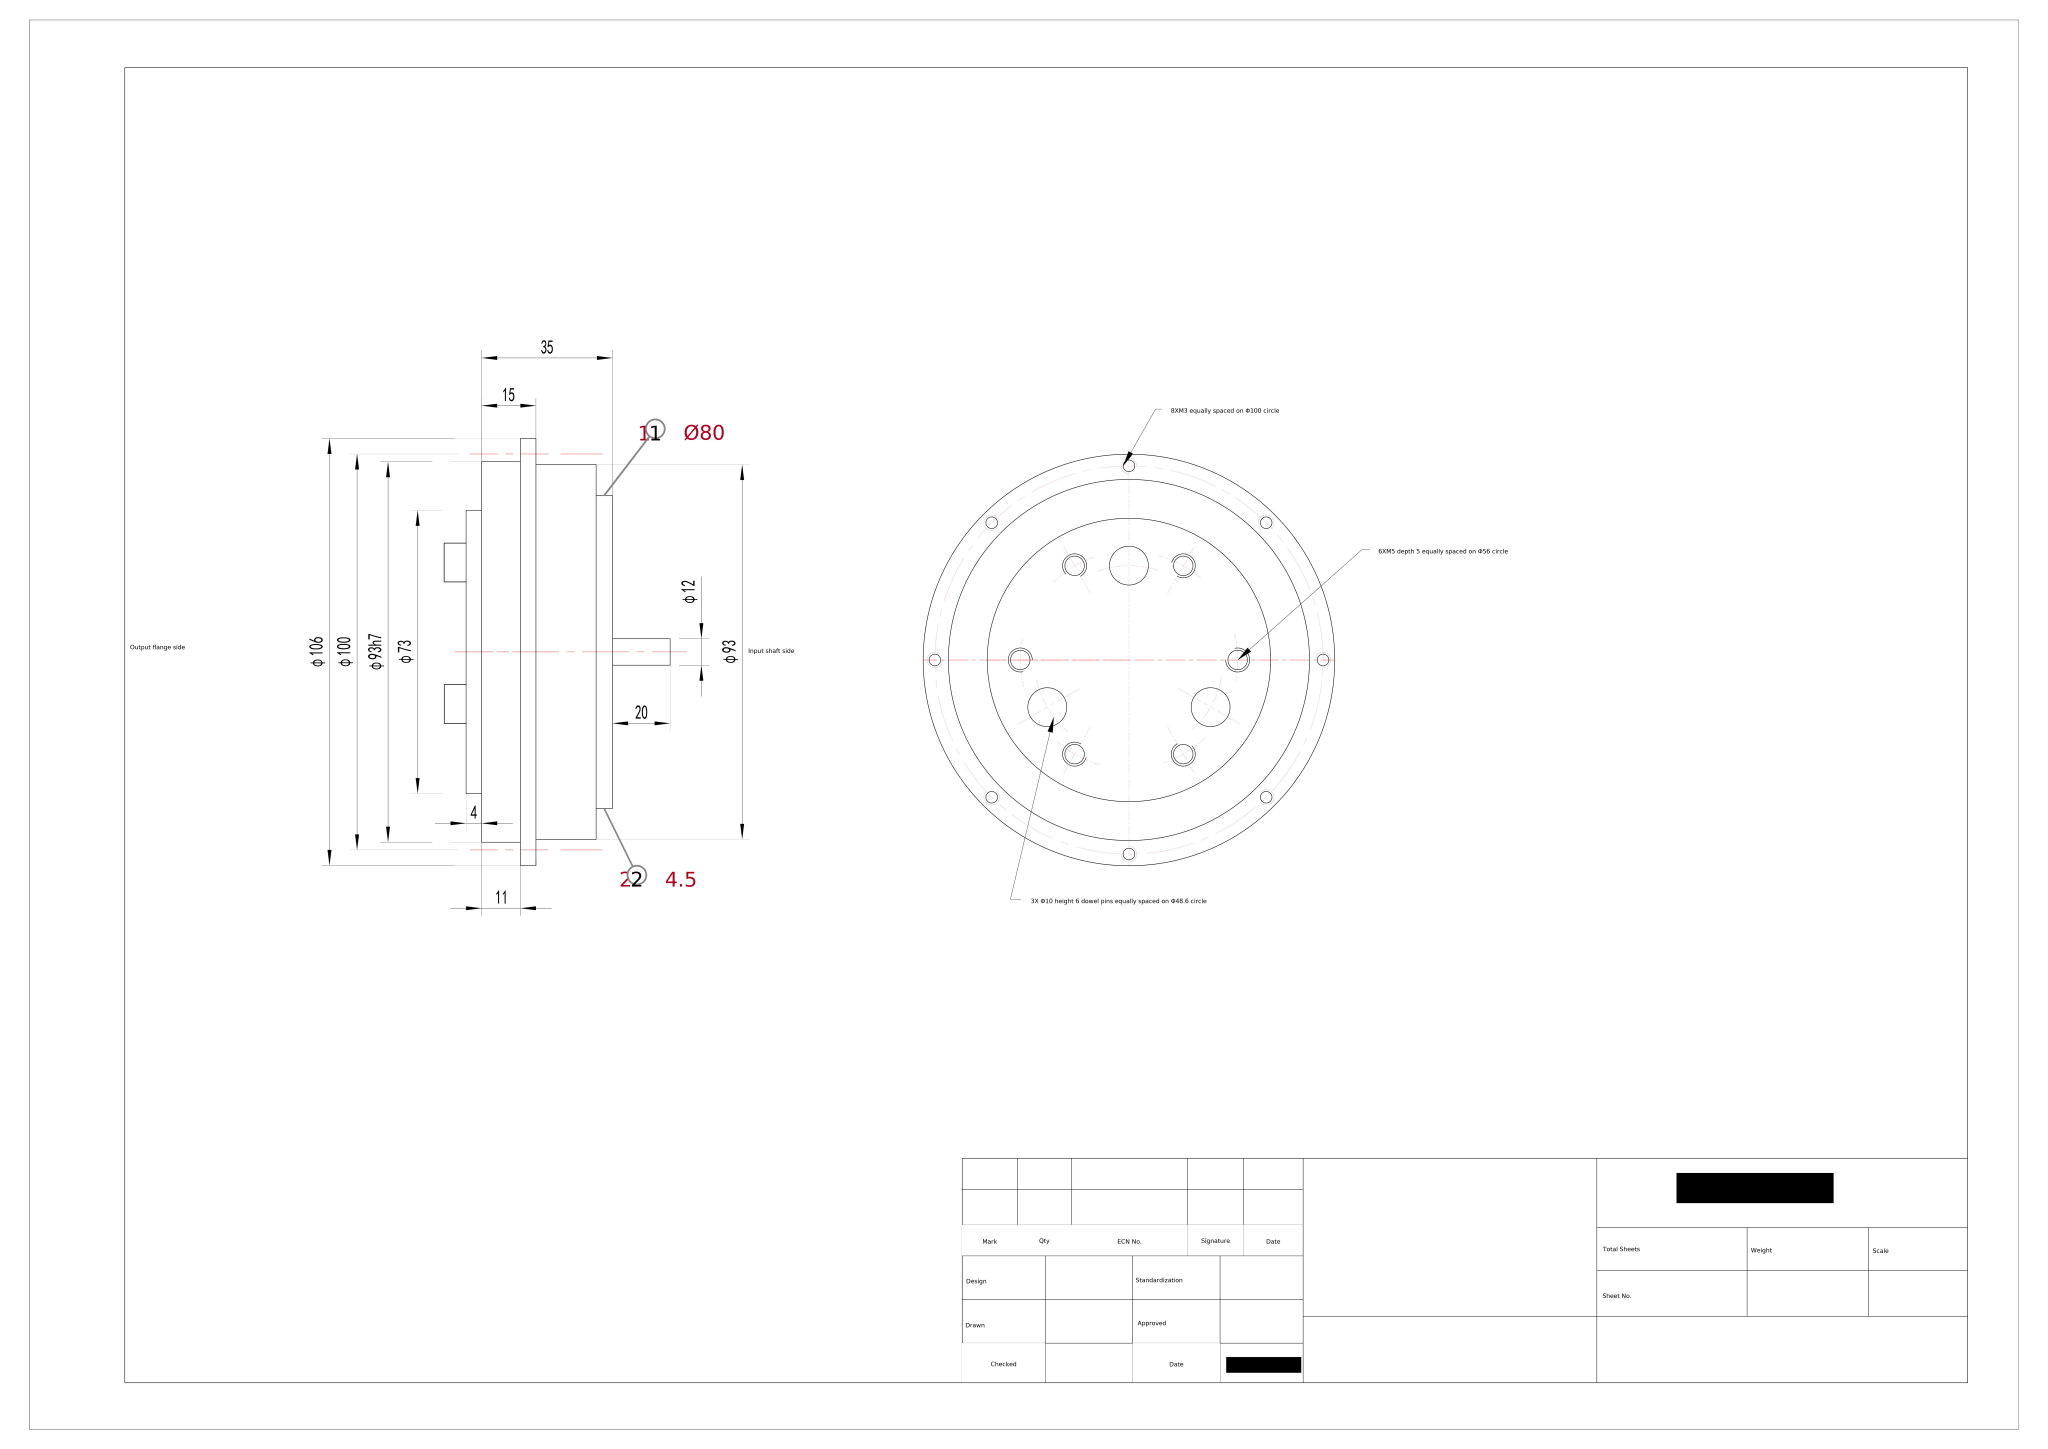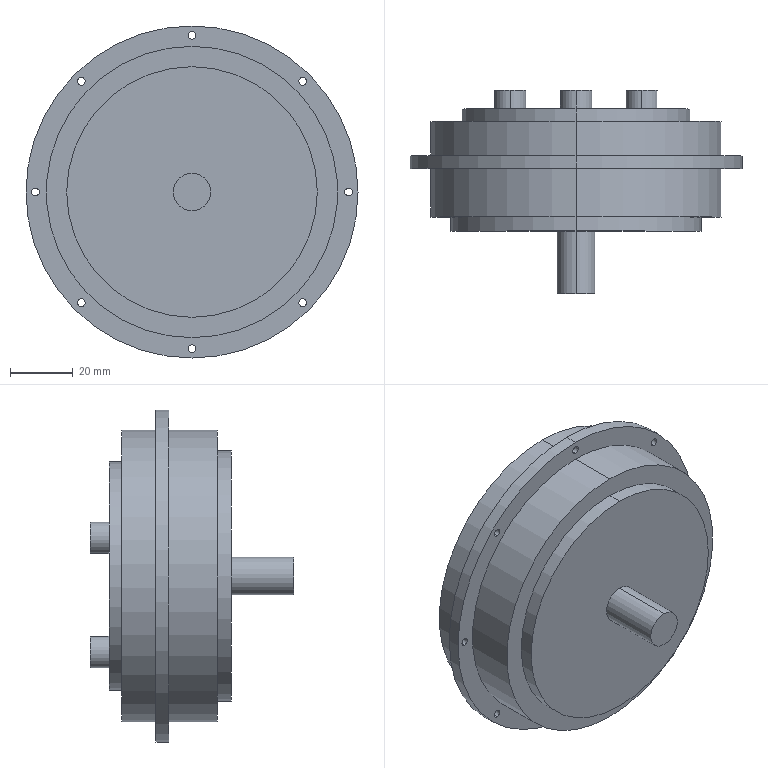Part | SolidWorks | mm | 1 solid | 96 faces | box 106 x 65 x 106 mm | volume 256982 mm3 | cylinder 46 | cone 40 | plane 10 | commonest cylinder face diameters 2.5 x16 4.2 x12 10 x6 93 x4 12 x2 80 x2 106 x2 73 x2
build123d program:
from build123d import *

# Parameters (mm, degrees)
SKETCH1_R                   = 36.5
BOSS_EXTRUDE1_DEPTH         = 4
SKETCH2_R                   = 5
BOSS_EXTRUDE2_DEPTH         = 6
SKETCH3_R                   = 46.5
BOSS_EXTRUDE3_DEPTH         = 11
SKETCH4_R                   = 53
BOSS_EXTRUDE4_DEPTH         = 4
SKETCH5_R                   = 46.5
BOSS_EXTRUDE5_DEPTH         = 15.5
SKETCH6_R                   = 40
BOSS_EXTRUDE6_DEPTH         = 4.5
SKETCH7_R                   = 6
BOSS_EXTRUDE7_DEPTH         = 20
M3_TAPPED_HOLE1_D           = 2.5
M3_TAPPED_HOLE1_DEPTH       = 8.5
M3_TAPPED_HOLE1_CSINK_D     = 3.05
M3_TAPPED_HOLE1_CSINK_ANGLE = 90
M3_TAPPED_HOLE1_TIP         = 0.7511
M5_TAPPED_HOLE1_D           = 4.2
M5_TAPPED_HOLE1_DEPTH       = 14
M5_TAPPED_HOLE1_CSINK_D     = 5.05
M5_TAPPED_HOLE1_CSINK_ANGLE = 90
M5_TAPPED_HOLE1_TIP         = 1.262


with BuildPart() as part:
    # Sketch1 → Boss-Extrude1 (new body)
    with BuildSketch(Plane(origin=(0, 0, 0), x_dir=(1, 0, 0), z_dir=(0, 1, 0))):
        with Locations(Location((0, 0, 0), (0, 0, 270))):
            Circle(SKETCH1_R)
    extrude(amount=BOSS_EXTRUDE1_DEPTH)

    # Sketch2 → Boss-Extrude2 (add)
    with BuildSketch(Plane(origin=(0, 4, 0), x_dir=(1, 0, 0), z_dir=(0, 1, 0))):
        with Locations(Location((0, 24.3, 0), (0, 0, 270))):
            Circle(SKETCH2_R)
        with Locations(Location((21.044, -12.15, 0), (0, 0, 270))):
            Circle(SKETCH2_R)
        with Locations(Location((-21.044, -12.15, 0), (0, 0, 270))):
            Circle(SKETCH2_R)
    extrude(amount=BOSS_EXTRUDE2_DEPTH)

    # Sketch3 → Boss-Extrude3 (add)
    with BuildSketch(Plane.XZ):
        with Locations(Location((0, 0, 0), (0, 0, 270))):
            Circle(SKETCH3_R)
    extrude(amount=BOSS_EXTRUDE3_DEPTH)

    # Sketch4 → Boss-Extrude4 (add)
    with BuildSketch(Plane.XZ.offset(11)):
        with Locations(Location((0, 0, 0), (0, 0, 270))):
            Circle(SKETCH4_R)
    extrude(amount=BOSS_EXTRUDE4_DEPTH)

    # Sketch5 → Boss-Extrude5 (add)
    with BuildSketch(Plane.XZ.offset(15)):
        with Locations(Location((0, 0, 0), (0, 0, 270))):
            Circle(SKETCH5_R)
    extrude(amount=BOSS_EXTRUDE5_DEPTH)

    # Sketch6 → Boss-Extrude6 (add)
    with BuildSketch(Plane.XZ.offset(30.5)):
        with Locations(Location((0, 0, 0), (0, 0, 270))):
            Circle(SKETCH6_R)
    extrude(amount=BOSS_EXTRUDE6_DEPTH)

    # Sketch7 → Boss-Extrude7 (add)
    with BuildSketch(Plane.XZ.offset(35)):
        with Locations(Location((0, 0, 0), (0, 0, 270))):
            Circle(SKETCH7_R)
    extrude(amount=BOSS_EXTRUDE7_DEPTH)

    # M3 Tapped Hole1
    with Locations(Plane(origin=(0, -11, 0), x_dir=(1, 0, 0), z_dir=(0, 1, 0))):
        with Locations((-35.355, 35.355), (0, 50), (35.355, 35.355), (50, 0), (35.355, -35.355), (0, -50), (-35.355, -35.355), (-50, 0)):
            CounterSinkHole(M3_TAPPED_HOLE1_D / 2, M3_TAPPED_HOLE1_CSINK_D / 2, depth=M3_TAPPED_HOLE1_DEPTH, counter_sink_angle=M3_TAPPED_HOLE1_CSINK_ANGLE)
            with Locations((0, 0, -(M3_TAPPED_HOLE1_DEPTH + M3_TAPPED_HOLE1_TIP / 2))):  # 118° drill point
                Cone(0, M3_TAPPED_HOLE1_D / 2, M3_TAPPED_HOLE1_TIP, mode=Mode.SUBTRACT)

    # M5 Tapped Hole1
    with Locations(Plane(origin=(0, 4, 0), x_dir=(1, 0, 0), z_dir=(0, 1, 0))):
        with Locations((28, 0), (14, -24.249), (-14, -24.249), (-28, 0), (-14, 24.249), (14, 24.249)):
            CounterSinkHole(M5_TAPPED_HOLE1_D / 2, M5_TAPPED_HOLE1_CSINK_D / 2, depth=M5_TAPPED_HOLE1_DEPTH, counter_sink_angle=M5_TAPPED_HOLE1_CSINK_ANGLE)
            with Locations((0, 0, -(M5_TAPPED_HOLE1_DEPTH + M5_TAPPED_HOLE1_TIP / 2))):  # 118° drill point
                Cone(0, M5_TAPPED_HOLE1_D / 2, M5_TAPPED_HOLE1_TIP, mode=Mode.SUBTRACT)


solid = part.part